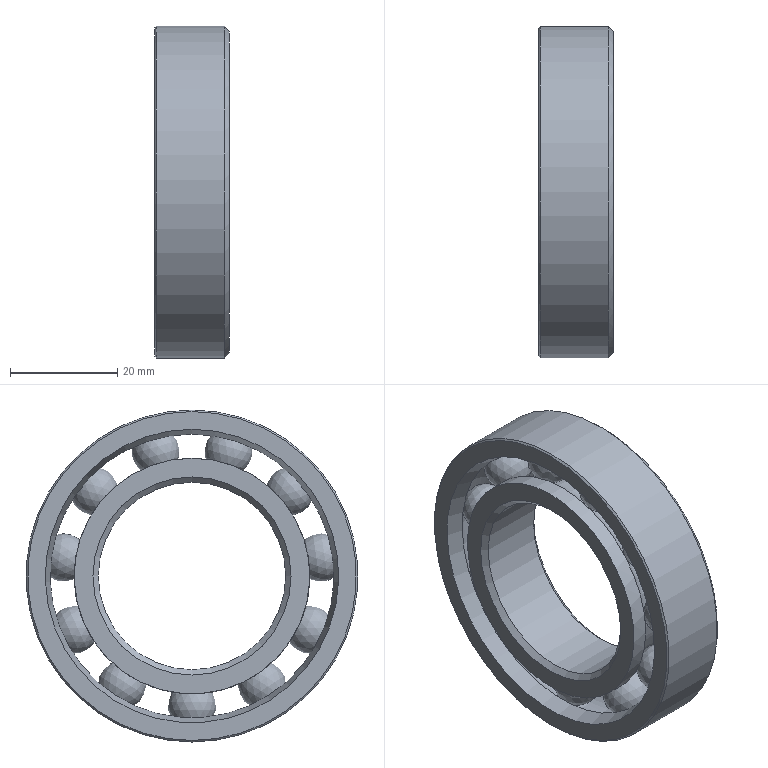Component | NX | GB-T292_AC-1994_7007_AC | 13 solids | 27 faces | volume 19155 mm3 | sphere 11 | cylinder 5 | cone 5 | plane 4 | torus 2 | commonest cylinder face diameters 44.001 x2 62 x1 52.999 x1 35 x1